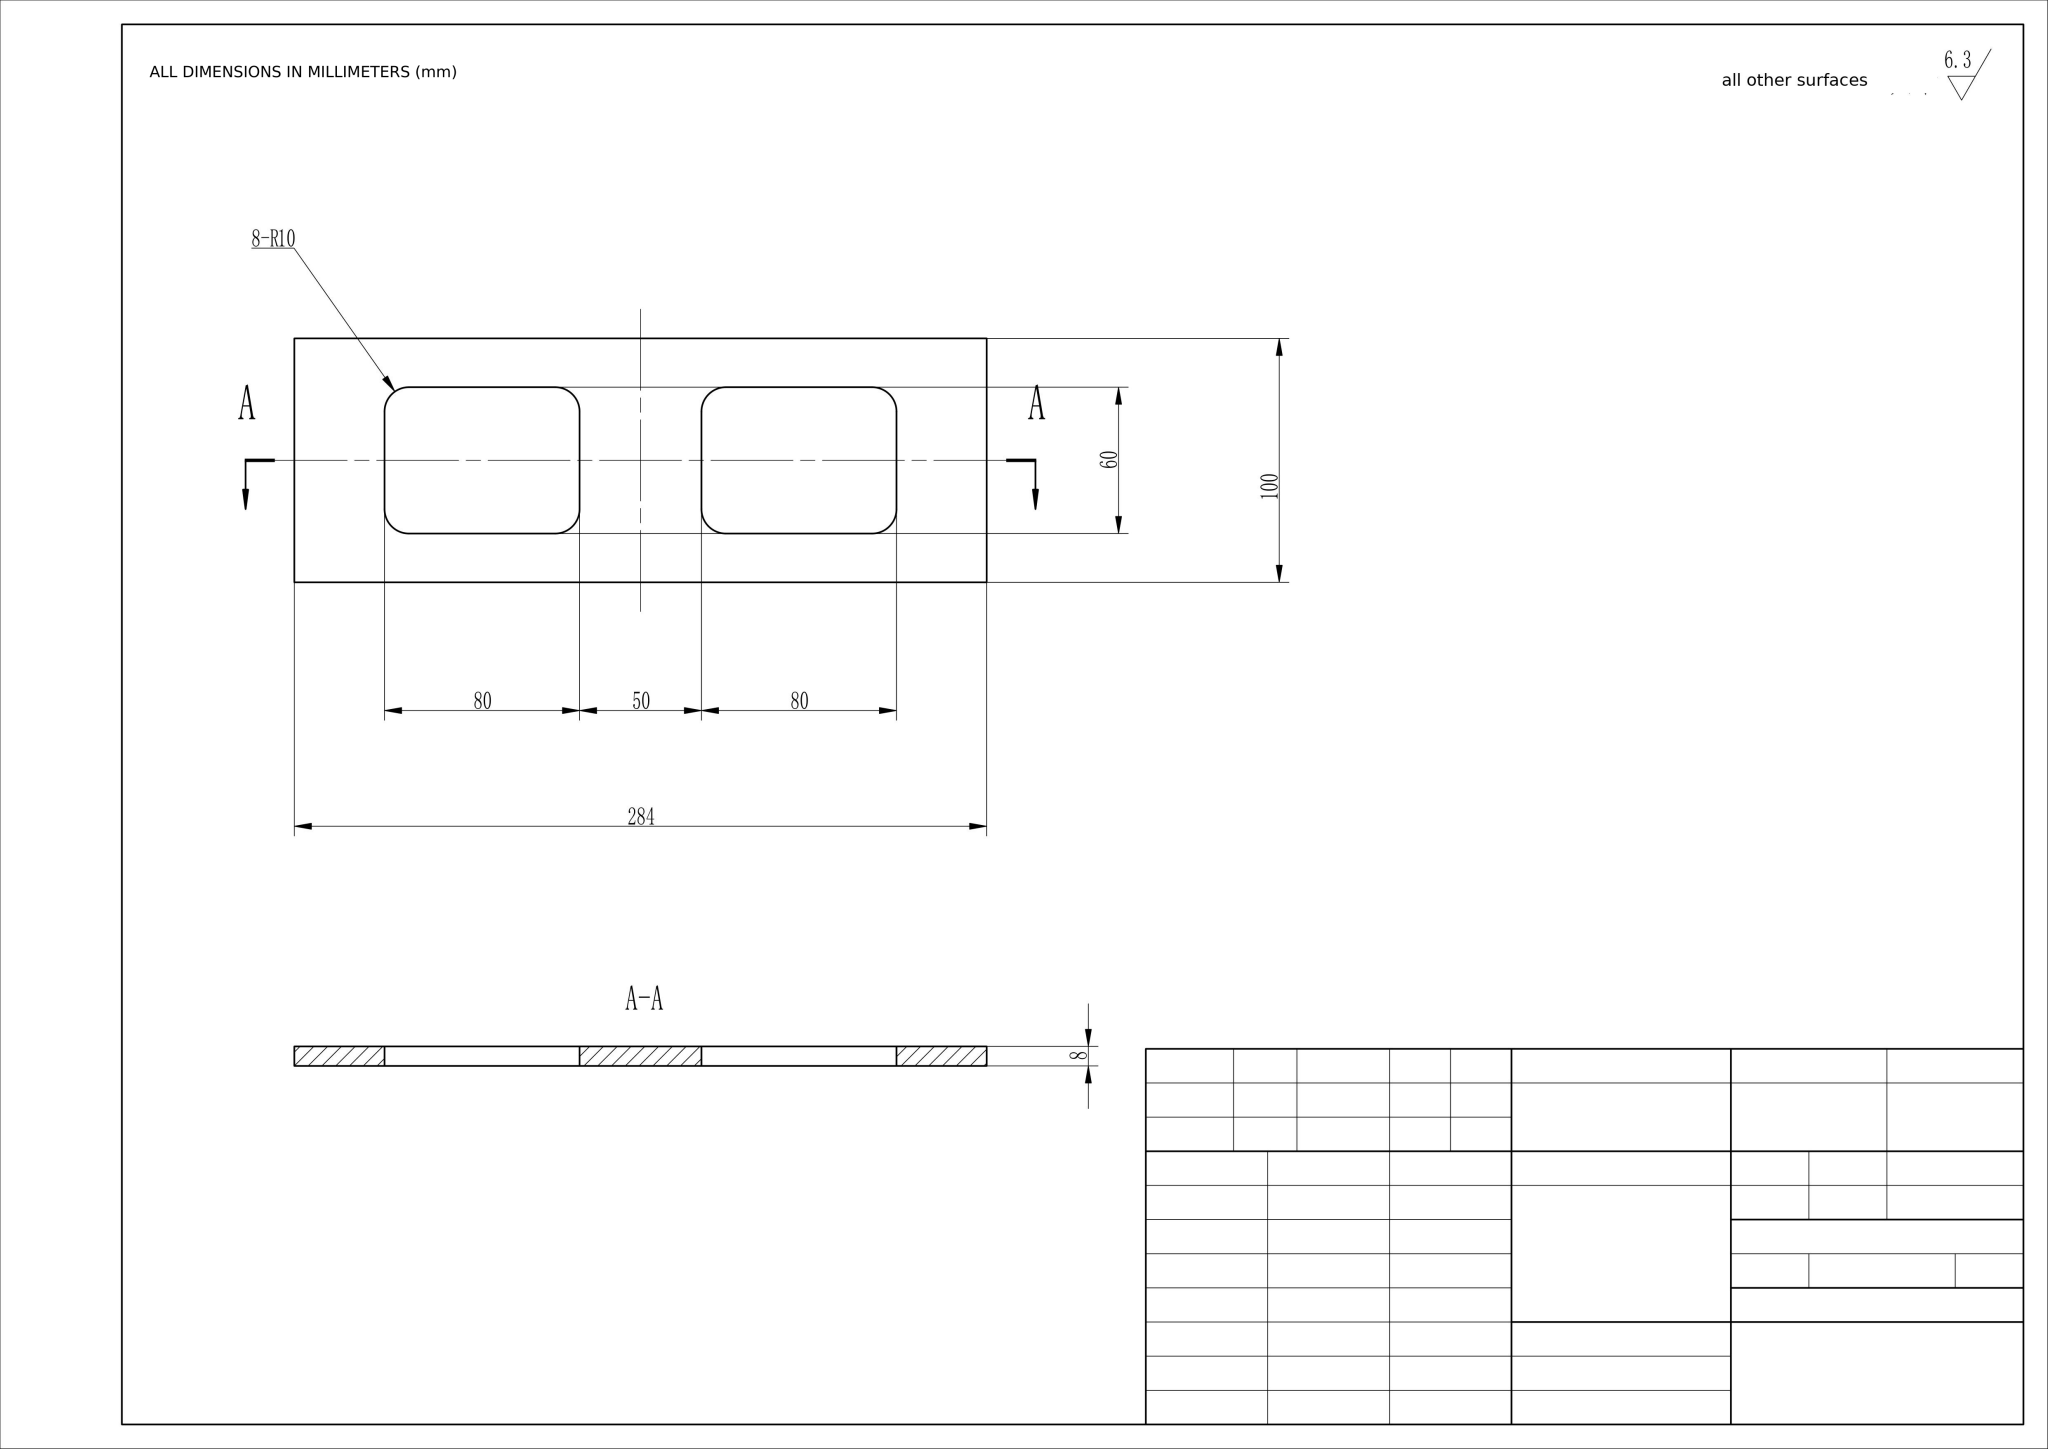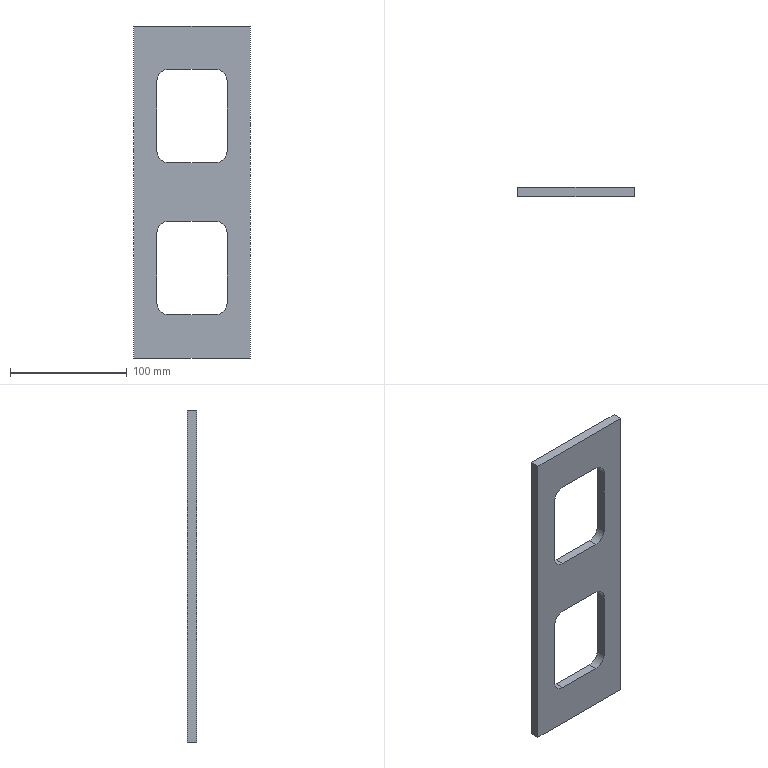Part | NX | mm | 1 solid | 22 faces | box 100 x 8 x 284 mm | volume 151773 mm3 | plane 14 | cylinder 8 | commonest cylinder face diameters 20 x8
STEP:
#1=CARTESIAN_POINT('',(0.,0.,0.));
#2=DIRECTION('',(0.,0.,1.));
#3=DIRECTION('',(1.,0.,0.));
#4=AXIS2_PLACEMENT_3D('',#1,#2,#3);
#5=(LENGTH_UNIT()NAMED_UNIT(*)SI_UNIT(.MILLI.,.METRE.));
#6=UNCERTAINTY_MEASURE_WITH_UNIT(LENGTH_MEASURE(0.00002),#5,'','');
#7=(NAMED_UNIT(*)PLANE_ANGLE_UNIT()SI_UNIT($,.RADIAN.));
#8=PLANE_ANGLE_MEASURE_WITH_UNIT(PLANE_ANGLE_MEASURE(0.01745),#7);
#9=DIMENSIONAL_EXPONENTS(0.,0.,0.,0.,0.,0.,0.);
#10=(CONVERSION_BASED_UNIT('',#8)NAMED_UNIT(#9)PLANE_ANGLE_UNIT());
#11=(NAMED_UNIT(*)SI_UNIT($,.STERADIAN.)SOLID_ANGLE_UNIT());
#12=(GEOMETRIC_REPRESENTATION_CONTEXT(3)GLOBAL_UNCERTAINTY_ASSIGNED_CONTEXT((#6))GLOBAL_UNIT_ASSIGNED_CONTEXT((#5,#10,#11))REPRESENTATION_CONTEXT('',''));
#13=SHAPE_REPRESENTATION('',(#4),#12);
#14=CARTESIAN_POINT('',(-0.,-8.,284.));
#15=VERTEX_POINT('',#14);
#16=CARTESIAN_POINT('',(0.,-8.,0.));
#17=VERTEX_POINT('',#16);
#18=CARTESIAN_POINT('',(-0.,-8.,284.));
#19=DIRECTION('',(0.,0.,-1.));
#20=VECTOR('',#19,1.);
#21=LINE('',#18,#20);
#22=EDGE_CURVE('',#15,#17,#21,.T.);
#23=ORIENTED_EDGE('',*,*,#22,.T.);
#24=CARTESIAN_POINT('',(100.,-8.,0.));
#25=VERTEX_POINT('',#24);
#26=CARTESIAN_POINT('',(0.,-8.,0.));
#27=DIRECTION('',(1.,0.,0.));
#28=VECTOR('',#27,1.);
#29=LINE('',#26,#28);
#30=EDGE_CURVE('',#17,#25,#29,.T.);
#31=ORIENTED_EDGE('',*,*,#30,.T.);
#32=CARTESIAN_POINT('',(100.,-8.,284.));
#33=VERTEX_POINT('',#32);
#34=CARTESIAN_POINT('',(100.,-8.,0.));
#35=DIRECTION('',(-0.,0.,1.));
#36=VECTOR('',#35,1.);
#37=LINE('',#34,#36);
#38=EDGE_CURVE('',#25,#33,#37,.T.);
#39=ORIENTED_EDGE('',*,*,#38,.T.);
#40=CARTESIAN_POINT('',(100.,-8.,284.));
#41=DIRECTION('',(-1.,0.,0.));
#42=VECTOR('',#41,1.);
#43=LINE('',#40,#42);
#44=EDGE_CURVE('',#33,#15,#43,.T.);
#45=ORIENTED_EDGE('',*,*,#44,.T.);
#46=EDGE_LOOP('',(#23,#31,#39,#45));
#47=FACE_BOUND('',#46,.T.);
#48=CARTESIAN_POINT('',(80.,-8.,237.));
#49=VERTEX_POINT('',#48);
#50=CARTESIAN_POINT('',(80.,-8.,177.));
#51=VERTEX_POINT('',#50);
#52=CARTESIAN_POINT('',(80.,-8.,247.));
#53=DIRECTION('',(0.,0.,-1.));
#54=VECTOR('',#53,1.);
#55=LINE('',#52,#54);
#56=EDGE_CURVE('',#49,#51,#55,.T.);
#57=ORIENTED_EDGE('',*,*,#56,.T.);
#58=CARTESIAN_POINT('',(70.,-8.,167.));
#59=VERTEX_POINT('',#58);
#60=CARTESIAN_POINT('',(70.,-8.,177.));
#61=DIRECTION('',(0.,1.,0.));
#62=DIRECTION('',(0.,0.,-1.));
#63=AXIS2_PLACEMENT_3D('',#60,#61,#62);
#64=CIRCLE('',#63,10.);
#65=EDGE_CURVE('',#51,#59,#64,.T.);
#66=ORIENTED_EDGE('',*,*,#65,.T.);
#67=CARTESIAN_POINT('',(30.,-8.,167.));
#68=VERTEX_POINT('',#67);
#69=CARTESIAN_POINT('',(80.,-8.,167.));
#70=DIRECTION('',(-1.,0.,0.));
#71=VECTOR('',#70,1.);
#72=LINE('',#69,#71);
#73=EDGE_CURVE('',#59,#68,#72,.T.);
#74=ORIENTED_EDGE('',*,*,#73,.T.);
#75=CARTESIAN_POINT('',(20.,-8.,177.));
#76=VERTEX_POINT('',#75);
#77=CARTESIAN_POINT('',(30.,-8.,177.));
#78=DIRECTION('',(0.,1.,0.));
#79=DIRECTION('',(0.,0.,-1.));
#80=AXIS2_PLACEMENT_3D('',#77,#78,#79);
#81=CIRCLE('',#80,10.);
#82=EDGE_CURVE('',#68,#76,#81,.T.);
#83=ORIENTED_EDGE('',*,*,#82,.T.);
#84=CARTESIAN_POINT('',(20.,-8.,237.));
#85=VERTEX_POINT('',#84);
#86=CARTESIAN_POINT('',(20.,-8.,167.));
#87=DIRECTION('',(0.,0.,1.));
#88=VECTOR('',#87,1.);
#89=LINE('',#86,#88);
#90=EDGE_CURVE('',#76,#85,#89,.T.);
#91=ORIENTED_EDGE('',*,*,#90,.T.);
#92=CARTESIAN_POINT('',(30.,-8.,247.));
#93=VERTEX_POINT('',#92);
#94=CARTESIAN_POINT('',(30.,-8.,237.));
#95=DIRECTION('',(0.,1.,0.));
#96=DIRECTION('',(0.,0.,-1.));
#97=AXIS2_PLACEMENT_3D('',#94,#95,#96);
#98=CIRCLE('',#97,10.);
#99=EDGE_CURVE('',#85,#93,#98,.T.);
#100=ORIENTED_EDGE('',*,*,#99,.T.);
#101=CARTESIAN_POINT('',(70.,-8.,247.));
#102=VERTEX_POINT('',#101);
#103=CARTESIAN_POINT('',(20.,-8.,247.));
#104=DIRECTION('',(1.,0.,0.));
#105=VECTOR('',#104,1.);
#106=LINE('',#103,#105);
#107=EDGE_CURVE('',#93,#102,#106,.T.);
#108=ORIENTED_EDGE('',*,*,#107,.T.);
#109=CARTESIAN_POINT('',(70.,-8.,237.));
#110=DIRECTION('',(0.,1.,0.));
#111=DIRECTION('',(0.,0.,-1.));
#112=AXIS2_PLACEMENT_3D('',#109,#110,#111);
#113=CIRCLE('',#112,10.);
#114=EDGE_CURVE('',#102,#49,#113,.T.);
#115=ORIENTED_EDGE('',*,*,#114,.T.);
#116=EDGE_LOOP('',(#57,#66,#74,#83,#91,#100,#108,#115));
#117=FACE_BOUND('',#116,.T.);
#118=CARTESIAN_POINT('',(80.,-8.,107.));
#119=VERTEX_POINT('',#118);
#120=CARTESIAN_POINT('',(80.,-8.,47.));
#121=VERTEX_POINT('',#120);
#122=CARTESIAN_POINT('',(80.,-8.,117.));
#123=DIRECTION('',(-0.,0.,-1.));
#124=VECTOR('',#123,1.);
#125=LINE('',#122,#124);
#126=EDGE_CURVE('',#119,#121,#125,.T.);
#127=ORIENTED_EDGE('',*,*,#126,.T.);
#128=CARTESIAN_POINT('',(70.,-8.,37.));
#129=VERTEX_POINT('',#128);
#130=CARTESIAN_POINT('',(70.,-8.,47.));
#131=DIRECTION('',(0.,1.,0.));
#132=DIRECTION('',(0.,0.,-1.));
#133=AXIS2_PLACEMENT_3D('',#130,#131,#132);
#134=CIRCLE('',#133,10.);
#135=EDGE_CURVE('',#121,#129,#134,.T.);
#136=ORIENTED_EDGE('',*,*,#135,.T.);
#137=CARTESIAN_POINT('',(30.,-8.,37.));
#138=VERTEX_POINT('',#137);
#139=CARTESIAN_POINT('',(80.,-8.,37.));
#140=DIRECTION('',(-1.,0.,0.));
#141=VECTOR('',#140,1.);
#142=LINE('',#139,#141);
#143=EDGE_CURVE('',#129,#138,#142,.T.);
#144=ORIENTED_EDGE('',*,*,#143,.T.);
#145=CARTESIAN_POINT('',(20.,-8.,47.));
#146=VERTEX_POINT('',#145);
#147=CARTESIAN_POINT('',(30.,-8.,47.));
#148=DIRECTION('',(0.,1.,0.));
#149=DIRECTION('',(0.,0.,-1.));
#150=AXIS2_PLACEMENT_3D('',#147,#148,#149);
#151=CIRCLE('',#150,10.);
#152=EDGE_CURVE('',#138,#146,#151,.T.);
#153=ORIENTED_EDGE('',*,*,#152,.T.);
#154=CARTESIAN_POINT('',(20.,-8.,107.));
#155=VERTEX_POINT('',#154);
#156=CARTESIAN_POINT('',(20.,-8.,37.));
#157=DIRECTION('',(-0.,0.,1.));
#158=VECTOR('',#157,1.);
#159=LINE('',#156,#158);
#160=EDGE_CURVE('',#146,#155,#159,.T.);
#161=ORIENTED_EDGE('',*,*,#160,.T.);
#162=CARTESIAN_POINT('',(30.,-8.,117.));
#163=VERTEX_POINT('',#162);
#164=CARTESIAN_POINT('',(30.,-8.,107.));
#165=DIRECTION('',(0.,1.,0.));
#166=DIRECTION('',(0.,0.,-1.));
#167=AXIS2_PLACEMENT_3D('',#164,#165,#166);
#168=CIRCLE('',#167,10.);
#169=EDGE_CURVE('',#155,#163,#168,.T.);
#170=ORIENTED_EDGE('',*,*,#169,.T.);
#171=CARTESIAN_POINT('',(70.,-8.,117.));
#172=VERTEX_POINT('',#171);
#173=CARTESIAN_POINT('',(20.,-8.,117.));
#174=DIRECTION('',(1.,0.,0.));
#175=VECTOR('',#174,1.);
#176=LINE('',#173,#175);
#177=EDGE_CURVE('',#163,#172,#176,.T.);
#178=ORIENTED_EDGE('',*,*,#177,.T.);
#179=CARTESIAN_POINT('',(70.,-8.,107.));
#180=DIRECTION('',(0.,1.,0.));
#181=DIRECTION('',(0.,0.,-1.));
#182=AXIS2_PLACEMENT_3D('',#179,#180,#181);
#183=CIRCLE('',#182,10.);
#184=EDGE_CURVE('',#172,#119,#183,.T.);
#185=ORIENTED_EDGE('',*,*,#184,.T.);
#186=EDGE_LOOP('',(#127,#136,#144,#153,#161,#170,#178,#185));
#187=FACE_BOUND('',#186,.T.);
#188=CARTESIAN_POINT('',(0.,-8.,0.));
#189=DIRECTION('',(0.,-1.,0.));
#190=DIRECTION('',(0.,0.,-1.));
#191=AXIS2_PLACEMENT_3D('',#188,#189,#190);
#192=PLANE('',#191);
#193=ADVANCED_FACE('',(#47,#117,#187),#192,.T.);
#194=CARTESIAN_POINT('',(20.,0.,177.));
#195=VERTEX_POINT('',#194);
#196=CARTESIAN_POINT('',(20.,0.,237.));
#197=VERTEX_POINT('',#196);
#198=CARTESIAN_POINT('',(20.,0.,167.));
#199=DIRECTION('',(0.,0.,1.));
#200=VECTOR('',#199,1.);
#201=LINE('',#198,#200);
#202=EDGE_CURVE('',#195,#197,#201,.T.);
#203=ORIENTED_EDGE('',*,*,#202,.F.);
#204=CARTESIAN_POINT('',(30.,0.,167.));
#205=VERTEX_POINT('',#204);
#206=CARTESIAN_POINT('',(30.,0.,177.));
#207=DIRECTION('',(0.,-1.,0.));
#208=DIRECTION('',(0.,0.,-1.));
#209=AXIS2_PLACEMENT_3D('',#206,#207,#208);
#210=CIRCLE('',#209,10.);
#211=EDGE_CURVE('',#195,#205,#210,.T.);
#212=ORIENTED_EDGE('',*,*,#211,.T.);
#213=CARTESIAN_POINT('',(70.,0.,167.));
#214=VERTEX_POINT('',#213);
#215=CARTESIAN_POINT('',(80.,0.,167.));
#216=DIRECTION('',(-1.,0.,0.));
#217=VECTOR('',#216,1.);
#218=LINE('',#215,#217);
#219=EDGE_CURVE('',#214,#205,#218,.T.);
#220=ORIENTED_EDGE('',*,*,#219,.F.);
#221=CARTESIAN_POINT('',(80.,0.,177.));
#222=VERTEX_POINT('',#221);
#223=CARTESIAN_POINT('',(70.,0.,177.));
#224=DIRECTION('',(0.,-1.,0.));
#225=DIRECTION('',(0.,0.,-1.));
#226=AXIS2_PLACEMENT_3D('',#223,#224,#225);
#227=CIRCLE('',#226,10.);
#228=EDGE_CURVE('',#214,#222,#227,.T.);
#229=ORIENTED_EDGE('',*,*,#228,.T.);
#230=CARTESIAN_POINT('',(80.,0.,237.));
#231=VERTEX_POINT('',#230);
#232=CARTESIAN_POINT('',(80.,0.,247.));
#233=DIRECTION('',(0.,0.,-1.));
#234=VECTOR('',#233,1.);
#235=LINE('',#232,#234);
#236=EDGE_CURVE('',#231,#222,#235,.T.);
#237=ORIENTED_EDGE('',*,*,#236,.F.);
#238=CARTESIAN_POINT('',(70.,0.,247.));
#239=VERTEX_POINT('',#238);
#240=CARTESIAN_POINT('',(70.,0.,237.));
#241=DIRECTION('',(0.,-1.,0.));
#242=DIRECTION('',(0.,0.,-1.));
#243=AXIS2_PLACEMENT_3D('',#240,#241,#242);
#244=CIRCLE('',#243,10.);
#245=EDGE_CURVE('',#231,#239,#244,.T.);
#246=ORIENTED_EDGE('',*,*,#245,.T.);
#247=CARTESIAN_POINT('',(30.,0.,247.));
#248=VERTEX_POINT('',#247);
#249=CARTESIAN_POINT('',(20.,0.,247.));
#250=DIRECTION('',(1.,0.,0.));
#251=VECTOR('',#250,1.);
#252=LINE('',#249,#251);
#253=EDGE_CURVE('',#248,#239,#252,.T.);
#254=ORIENTED_EDGE('',*,*,#253,.F.);
#255=CARTESIAN_POINT('',(30.,0.,237.));
#256=DIRECTION('',(0.,-1.,0.));
#257=DIRECTION('',(0.,0.,-1.));
#258=AXIS2_PLACEMENT_3D('',#255,#256,#257);
#259=CIRCLE('',#258,10.);
#260=EDGE_CURVE('',#248,#197,#259,.T.);
#261=ORIENTED_EDGE('',*,*,#260,.T.);
#262=EDGE_LOOP('',(#203,#212,#220,#229,#237,#246,#254,#261));
#263=FACE_BOUND('',#262,.T.);
#264=CARTESIAN_POINT('',(-0.,0.,284.));
#265=VERTEX_POINT('',#264);
#266=CARTESIAN_POINT('',(0.,0.,0.));
#267=VERTEX_POINT('',#266);
#268=CARTESIAN_POINT('',(-0.,0.,284.));
#269=DIRECTION('',(0.,0.,-1.));
#270=VECTOR('',#269,1.);
#271=LINE('',#268,#270);
#272=EDGE_CURVE('',#265,#267,#271,.T.);
#273=ORIENTED_EDGE('',*,*,#272,.F.);
#274=CARTESIAN_POINT('',(100.,0.,284.));
#275=VERTEX_POINT('',#274);
#276=CARTESIAN_POINT('',(100.,0.,284.));
#277=DIRECTION('',(-1.,0.,0.));
#278=VECTOR('',#277,1.);
#279=LINE('',#276,#278);
#280=EDGE_CURVE('',#275,#265,#279,.T.);
#281=ORIENTED_EDGE('',*,*,#280,.F.);
#282=CARTESIAN_POINT('',(100.,0.,0.));
#283=VERTEX_POINT('',#282);
#284=CARTESIAN_POINT('',(100.,0.,0.));
#285=DIRECTION('',(-0.,0.,1.));
#286=VECTOR('',#285,1.);
#287=LINE('',#284,#286);
#288=EDGE_CURVE('',#283,#275,#287,.T.);
#289=ORIENTED_EDGE('',*,*,#288,.F.);
#290=CARTESIAN_POINT('',(0.,0.,0.));
#291=DIRECTION('',(1.,0.,0.));
#292=VECTOR('',#291,1.);
#293=LINE('',#290,#292);
#294=EDGE_CURVE('',#267,#283,#293,.T.);
#295=ORIENTED_EDGE('',*,*,#294,.F.);
#296=EDGE_LOOP('',(#273,#281,#289,#295));
#297=FACE_BOUND('',#296,.T.);
#298=CARTESIAN_POINT('',(20.,0.,47.));
#299=VERTEX_POINT('',#298);
#300=CARTESIAN_POINT('',(20.,0.,107.));
#301=VERTEX_POINT('',#300);
#302=CARTESIAN_POINT('',(20.,0.,37.));
#303=DIRECTION('',(-0.,0.,1.));
#304=VECTOR('',#303,1.);
#305=LINE('',#302,#304);
#306=EDGE_CURVE('',#299,#301,#305,.T.);
#307=ORIENTED_EDGE('',*,*,#306,.F.);
#308=CARTESIAN_POINT('',(30.,0.,37.));
#309=VERTEX_POINT('',#308);
#310=CARTESIAN_POINT('',(30.,0.,47.));
#311=DIRECTION('',(0.,-1.,0.));
#312=DIRECTION('',(0.,0.,-1.));
#313=AXIS2_PLACEMENT_3D('',#310,#311,#312);
#314=CIRCLE('',#313,10.);
#315=EDGE_CURVE('',#299,#309,#314,.T.);
#316=ORIENTED_EDGE('',*,*,#315,.T.);
#317=CARTESIAN_POINT('',(70.,0.,37.));
#318=VERTEX_POINT('',#317);
#319=CARTESIAN_POINT('',(80.,0.,37.));
#320=DIRECTION('',(-1.,0.,0.));
#321=VECTOR('',#320,1.);
#322=LINE('',#319,#321);
#323=EDGE_CURVE('',#318,#309,#322,.T.);
#324=ORIENTED_EDGE('',*,*,#323,.F.);
#325=CARTESIAN_POINT('',(80.,0.,47.));
#326=VERTEX_POINT('',#325);
#327=CARTESIAN_POINT('',(70.,0.,47.));
#328=DIRECTION('',(0.,-1.,0.));
#329=DIRECTION('',(0.,0.,-1.));
#330=AXIS2_PLACEMENT_3D('',#327,#328,#329);
#331=CIRCLE('',#330,10.);
#332=EDGE_CURVE('',#318,#326,#331,.T.);
#333=ORIENTED_EDGE('',*,*,#332,.T.);
#334=CARTESIAN_POINT('',(80.,0.,107.));
#335=VERTEX_POINT('',#334);
#336=CARTESIAN_POINT('',(80.,0.,117.));
#337=DIRECTION('',(-0.,0.,-1.));
#338=VECTOR('',#337,1.);
#339=LINE('',#336,#338);
#340=EDGE_CURVE('',#335,#326,#339,.T.);
#341=ORIENTED_EDGE('',*,*,#340,.F.);
#342=CARTESIAN_POINT('',(70.,0.,117.));
#343=VERTEX_POINT('',#342);
#344=CARTESIAN_POINT('',(70.,0.,107.));
#345=DIRECTION('',(0.,-1.,0.));
#346=DIRECTION('',(0.,0.,-1.));
#347=AXIS2_PLACEMENT_3D('',#344,#345,#346);
#348=CIRCLE('',#347,10.);
#349=EDGE_CURVE('',#335,#343,#348,.T.);
#350=ORIENTED_EDGE('',*,*,#349,.T.);
#351=CARTESIAN_POINT('',(30.,0.,117.));
#352=VERTEX_POINT('',#351);
#353=CARTESIAN_POINT('',(20.,0.,117.));
#354=DIRECTION('',(1.,0.,0.));
#355=VECTOR('',#354,1.);
#356=LINE('',#353,#355);
#357=EDGE_CURVE('',#352,#343,#356,.T.);
#358=ORIENTED_EDGE('',*,*,#357,.F.);
#359=CARTESIAN_POINT('',(30.,0.,107.));
#360=DIRECTION('',(0.,-1.,0.));
#361=DIRECTION('',(0.,0.,-1.));
#362=AXIS2_PLACEMENT_3D('',#359,#360,#361);
#363=CIRCLE('',#362,10.);
#364=EDGE_CURVE('',#352,#301,#363,.T.);
#365=ORIENTED_EDGE('',*,*,#364,.T.);
#366=EDGE_LOOP('',(#307,#316,#324,#333,#341,#350,#358,#365));
#367=FACE_BOUND('',#366,.T.);
#368=CARTESIAN_POINT('',(0.,0.,0.));
#369=DIRECTION('',(0.,-1.,0.));
#370=DIRECTION('',(0.,0.,-1.));
#371=AXIS2_PLACEMENT_3D('',#368,#369,#370);
#372=PLANE('',#371);
#373=ADVANCED_FACE('',(#263,#297,#367),#372,.F.);
#374=ORIENTED_EDGE('',*,*,#272,.T.);
#375=CARTESIAN_POINT('',(0.,-8.,0.));
#376=DIRECTION('',(0.,1.,0.));
#377=VECTOR('',#376,1.);
#378=LINE('',#375,#377);
#379=EDGE_CURVE('',#17,#267,#378,.T.);
#380=ORIENTED_EDGE('',*,*,#379,.F.);
#381=ORIENTED_EDGE('',*,*,#22,.F.);
#382=CARTESIAN_POINT('',(-0.,-8.,284.));
#383=DIRECTION('',(0.,1.,0.));
#384=VECTOR('',#383,1.);
#385=LINE('',#382,#384);
#386=EDGE_CURVE('',#15,#265,#385,.T.);
#387=ORIENTED_EDGE('',*,*,#386,.T.);
#388=EDGE_LOOP('',(#374,#380,#381,#387));
#389=FACE_OUTER_BOUND('',#388,.T.);
#390=CARTESIAN_POINT('',(-0.,-8.,284.));
#391=DIRECTION('',(1.,0.,0.));
#392=DIRECTION('',(0.,0.,-1.));
#393=AXIS2_PLACEMENT_3D('',#390,#391,#392);
#394=PLANE('',#393);
#395=ADVANCED_FACE('',(#389),#394,.F.);
#396=ORIENTED_EDGE('',*,*,#294,.T.);
#397=CARTESIAN_POINT('',(100.,-8.,0.));
#398=DIRECTION('',(0.,1.,0.));
#399=VECTOR('',#398,1.);
#400=LINE('',#397,#399);
#401=EDGE_CURVE('',#25,#283,#400,.T.);
#402=ORIENTED_EDGE('',*,*,#401,.F.);
#403=ORIENTED_EDGE('',*,*,#30,.F.);
#404=ORIENTED_EDGE('',*,*,#379,.T.);
#405=EDGE_LOOP('',(#396,#402,#403,#404));
#406=FACE_OUTER_BOUND('',#405,.T.);
#407=CARTESIAN_POINT('',(0.,-8.,0.));
#408=DIRECTION('',(0.,0.,1.));
#409=DIRECTION('',(1.,0.,0.));
#410=AXIS2_PLACEMENT_3D('',#407,#408,#409);
#411=PLANE('',#410);
#412=ADVANCED_FACE('',(#406),#411,.F.);
#413=ORIENTED_EDGE('',*,*,#288,.T.);
#414=CARTESIAN_POINT('',(100.,-8.,284.));
#415=DIRECTION('',(0.,1.,0.));
#416=VECTOR('',#415,1.);
#417=LINE('',#414,#416);
#418=EDGE_CURVE('',#33,#275,#417,.T.);
#419=ORIENTED_EDGE('',*,*,#418,.F.);
#420=ORIENTED_EDGE('',*,*,#38,.F.);
#421=ORIENTED_EDGE('',*,*,#401,.T.);
#422=EDGE_LOOP('',(#413,#419,#420,#421));
#423=FACE_OUTER_BOUND('',#422,.T.);
#424=CARTESIAN_POINT('',(100.,-8.,0.));
#425=DIRECTION('',(-1.,0.,-0.));
#426=DIRECTION('',(-0.,0.,1.));
#427=AXIS2_PLACEMENT_3D('',#424,#425,#426);
#428=PLANE('',#427);
#429=ADVANCED_FACE('',(#423),#428,.F.);
#430=ORIENTED_EDGE('',*,*,#280,.T.);
#431=ORIENTED_EDGE('',*,*,#386,.F.);
#432=ORIENTED_EDGE('',*,*,#44,.F.);
#433=ORIENTED_EDGE('',*,*,#418,.T.);
#434=EDGE_LOOP('',(#430,#431,#432,#433));
#435=FACE_OUTER_BOUND('',#434,.T.);
#436=CARTESIAN_POINT('',(100.,-8.,284.));
#437=DIRECTION('',(0.,0.,-1.));
#438=DIRECTION('',(-1.,0.,0.));
#439=AXIS2_PLACEMENT_3D('',#436,#437,#438);
#440=PLANE('',#439);
#441=ADVANCED_FACE('',(#435),#440,.F.);
#442=ORIENTED_EDGE('',*,*,#90,.F.);
#443=CARTESIAN_POINT('',(20.,0.,177.));
#444=DIRECTION('',(0.,1.,0.));
#445=VECTOR('',#444,1.);
#446=LINE('',#443,#445);
#447=EDGE_CURVE('',#76,#195,#446,.T.);
#448=ORIENTED_EDGE('',*,*,#447,.T.);
#449=ORIENTED_EDGE('',*,*,#202,.T.);
#450=CARTESIAN_POINT('',(20.,-8.,237.));
#451=DIRECTION('',(0.,-1.,0.));
#452=VECTOR('',#451,1.);
#453=LINE('',#450,#452);
#454=EDGE_CURVE('',#197,#85,#453,.T.);
#455=ORIENTED_EDGE('',*,*,#454,.T.);
#456=EDGE_LOOP('',(#442,#448,#449,#455));
#457=FACE_OUTER_BOUND('',#456,.T.);
#458=CARTESIAN_POINT('',(20.,-8.,167.));
#459=DIRECTION('',(-1.,0.,0.));
#460=DIRECTION('',(0.,0.,1.));
#461=AXIS2_PLACEMENT_3D('',#458,#459,#460);
#462=PLANE('',#461);
#463=ADVANCED_FACE('',(#457),#462,.F.);
#464=ORIENTED_EDGE('',*,*,#253,.T.);
#465=CARTESIAN_POINT('',(70.,-8.,247.));
#466=DIRECTION('',(0.,-1.,0.));
#467=VECTOR('',#466,1.);
#468=LINE('',#465,#467);
#469=EDGE_CURVE('',#239,#102,#468,.T.);
#470=ORIENTED_EDGE('',*,*,#469,.T.);
#471=ORIENTED_EDGE('',*,*,#107,.F.);
#472=CARTESIAN_POINT('',(30.,0.,247.));
#473=DIRECTION('',(0.,1.,0.));
#474=VECTOR('',#473,1.);
#475=LINE('',#472,#474);
#476=EDGE_CURVE('',#93,#248,#475,.T.);
#477=ORIENTED_EDGE('',*,*,#476,.T.);
#478=EDGE_LOOP('',(#464,#470,#471,#477));
#479=FACE_OUTER_BOUND('',#478,.T.);
#480=CARTESIAN_POINT('',(20.,-8.,247.));
#481=DIRECTION('',(0.,0.,1.));
#482=DIRECTION('',(1.,0.,0.));
#483=AXIS2_PLACEMENT_3D('',#480,#481,#482);
#484=PLANE('',#483);
#485=ADVANCED_FACE('',(#479),#484,.F.);
#486=ORIENTED_EDGE('',*,*,#236,.T.);
#487=CARTESIAN_POINT('',(80.,-8.,177.));
#488=DIRECTION('',(0.,-1.,0.));
#489=VECTOR('',#488,1.);
#490=LINE('',#487,#489);
#491=EDGE_CURVE('',#222,#51,#490,.T.);
#492=ORIENTED_EDGE('',*,*,#491,.T.);
#493=ORIENTED_EDGE('',*,*,#56,.F.);
#494=CARTESIAN_POINT('',(80.,0.,237.));
#495=DIRECTION('',(0.,1.,0.));
#496=VECTOR('',#495,1.);
#497=LINE('',#494,#496);
#498=EDGE_CURVE('',#49,#231,#497,.T.);
#499=ORIENTED_EDGE('',*,*,#498,.T.);
#500=EDGE_LOOP('',(#486,#492,#493,#499));
#501=FACE_OUTER_BOUND('',#500,.T.);
#502=CARTESIAN_POINT('',(80.,-8.,247.));
#503=DIRECTION('',(1.,0.,0.));
#504=DIRECTION('',(0.,0.,-1.));
#505=AXIS2_PLACEMENT_3D('',#502,#503,#504);
#506=PLANE('',#505);
#507=ADVANCED_FACE('',(#501),#506,.F.);
#508=ORIENTED_EDGE('',*,*,#73,.F.);
#509=CARTESIAN_POINT('',(70.,0.,167.));
#510=DIRECTION('',(0.,1.,0.));
#511=VECTOR('',#510,1.);
#512=LINE('',#509,#511);
#513=EDGE_CURVE('',#59,#214,#512,.T.);
#514=ORIENTED_EDGE('',*,*,#513,.T.);
#515=ORIENTED_EDGE('',*,*,#219,.T.);
#516=CARTESIAN_POINT('',(30.,-8.,167.));
#517=DIRECTION('',(0.,-1.,0.));
#518=VECTOR('',#517,1.);
#519=LINE('',#516,#518);
#520=EDGE_CURVE('',#205,#68,#519,.T.);
#521=ORIENTED_EDGE('',*,*,#520,.T.);
#522=EDGE_LOOP('',(#508,#514,#515,#521));
#523=FACE_OUTER_BOUND('',#522,.T.);
#524=CARTESIAN_POINT('',(80.,-8.,167.));
#525=DIRECTION('',(-0.,0.,-1.));
#526=DIRECTION('',(-1.,0.,0.));
#527=AXIS2_PLACEMENT_3D('',#524,#525,#526);
#528=PLANE('',#527);
#529=ADVANCED_FACE('',(#523),#528,.F.);
#530=ORIENTED_EDGE('',*,*,#160,.F.);
#531=CARTESIAN_POINT('',(20.,0.,47.));
#532=DIRECTION('',(0.,1.,0.));
#533=VECTOR('',#532,1.);
#534=LINE('',#531,#533);
#535=EDGE_CURVE('',#146,#299,#534,.T.);
#536=ORIENTED_EDGE('',*,*,#535,.T.);
#537=ORIENTED_EDGE('',*,*,#306,.T.);
#538=CARTESIAN_POINT('',(20.,-8.,107.));
#539=DIRECTION('',(0.,-1.,0.));
#540=VECTOR('',#539,1.);
#541=LINE('',#538,#540);
#542=EDGE_CURVE('',#301,#155,#541,.T.);
#543=ORIENTED_EDGE('',*,*,#542,.T.);
#544=EDGE_LOOP('',(#530,#536,#537,#543));
#545=FACE_OUTER_BOUND('',#544,.T.);
#546=CARTESIAN_POINT('',(20.,-8.,37.));
#547=DIRECTION('',(-1.,0.,-0.));
#548=DIRECTION('',(-0.,0.,1.));
#549=AXIS2_PLACEMENT_3D('',#546,#547,#548);
#550=PLANE('',#549);
#551=ADVANCED_FACE('',(#545),#550,.F.);
#552=ORIENTED_EDGE('',*,*,#357,.T.);
#553=CARTESIAN_POINT('',(70.,-8.,117.));
#554=DIRECTION('',(0.,-1.,0.));
#555=VECTOR('',#554,1.);
#556=LINE('',#553,#555);
#557=EDGE_CURVE('',#343,#172,#556,.T.);
#558=ORIENTED_EDGE('',*,*,#557,.T.);
#559=ORIENTED_EDGE('',*,*,#177,.F.);
#560=CARTESIAN_POINT('',(30.,0.,117.));
#561=DIRECTION('',(0.,1.,0.));
#562=VECTOR('',#561,1.);
#563=LINE('',#560,#562);
#564=EDGE_CURVE('',#163,#352,#563,.T.);
#565=ORIENTED_EDGE('',*,*,#564,.T.);
#566=EDGE_LOOP('',(#552,#558,#559,#565));
#567=FACE_OUTER_BOUND('',#566,.T.);
#568=CARTESIAN_POINT('',(20.,-8.,117.));
#569=DIRECTION('',(0.,0.,1.));
#570=DIRECTION('',(1.,0.,0.));
#571=AXIS2_PLACEMENT_3D('',#568,#569,#570);
#572=PLANE('',#571);
#573=ADVANCED_FACE('',(#567),#572,.F.);
#574=ORIENTED_EDGE('',*,*,#126,.F.);
#575=CARTESIAN_POINT('',(80.,0.,107.));
#576=DIRECTION('',(0.,1.,0.));
#577=VECTOR('',#576,1.);
#578=LINE('',#575,#577);
#579=EDGE_CURVE('',#119,#335,#578,.T.);
#580=ORIENTED_EDGE('',*,*,#579,.T.);
#581=ORIENTED_EDGE('',*,*,#340,.T.);
#582=CARTESIAN_POINT('',(80.,-8.,47.));
#583=DIRECTION('',(0.,-1.,0.));
#584=VECTOR('',#583,1.);
#585=LINE('',#582,#584);
#586=EDGE_CURVE('',#326,#121,#585,.T.);
#587=ORIENTED_EDGE('',*,*,#586,.T.);
#588=EDGE_LOOP('',(#574,#580,#581,#587));
#589=FACE_OUTER_BOUND('',#588,.T.);
#590=CARTESIAN_POINT('',(80.,-8.,117.));
#591=DIRECTION('',(1.,0.,-0.));
#592=DIRECTION('',(-0.,0.,-1.));
#593=AXIS2_PLACEMENT_3D('',#590,#591,#592);
#594=PLANE('',#593);
#595=ADVANCED_FACE('',(#589),#594,.F.);
#596=ORIENTED_EDGE('',*,*,#143,.F.);
#597=CARTESIAN_POINT('',(70.,0.,37.));
#598=DIRECTION('',(0.,1.,0.));
#599=VECTOR('',#598,1.);
#600=LINE('',#597,#599);
#601=EDGE_CURVE('',#129,#318,#600,.T.);
#602=ORIENTED_EDGE('',*,*,#601,.T.);
#603=ORIENTED_EDGE('',*,*,#323,.T.);
#604=CARTESIAN_POINT('',(30.,-8.,37.));
#605=DIRECTION('',(0.,-1.,0.));
#606=VECTOR('',#605,1.);
#607=LINE('',#604,#606);
#608=EDGE_CURVE('',#309,#138,#607,.T.);
#609=ORIENTED_EDGE('',*,*,#608,.T.);
#610=EDGE_LOOP('',(#596,#602,#603,#609));
#611=FACE_OUTER_BOUND('',#610,.T.);
#612=CARTESIAN_POINT('',(80.,-8.,37.));
#613=DIRECTION('',(0.,0.,-1.));
#614=DIRECTION('',(-1.,0.,0.));
#615=AXIS2_PLACEMENT_3D('',#612,#613,#614);
#616=PLANE('',#615);
#617=ADVANCED_FACE('',(#611),#616,.F.);
#618=ORIENTED_EDGE('',*,*,#228,.F.);
#619=ORIENTED_EDGE('',*,*,#513,.F.);
#620=ORIENTED_EDGE('',*,*,#65,.F.);
#621=ORIENTED_EDGE('',*,*,#491,.F.);
#622=EDGE_LOOP('',(#618,#619,#620,#621));
#623=FACE_OUTER_BOUND('',#622,.T.);
#624=CARTESIAN_POINT('',(70.,-8.,177.));
#625=DIRECTION('',(0.,1.,0.));
#626=DIRECTION('',(0.,0.,1.));
#627=AXIS2_PLACEMENT_3D('',#624,#625,#626);
#628=CYLINDRICAL_SURFACE('',#627,10.);
#629=ADVANCED_FACE('',(#623),#628,.F.);
#630=ORIENTED_EDGE('',*,*,#245,.F.);
#631=ORIENTED_EDGE('',*,*,#498,.F.);
#632=ORIENTED_EDGE('',*,*,#114,.F.);
#633=ORIENTED_EDGE('',*,*,#469,.F.);
#634=EDGE_LOOP('',(#630,#631,#632,#633));
#635=FACE_OUTER_BOUND('',#634,.T.);
#636=CARTESIAN_POINT('',(70.,-8.,237.));
#637=DIRECTION('',(0.,1.,0.));
#638=DIRECTION('',(0.,0.,1.));
#639=AXIS2_PLACEMENT_3D('',#636,#637,#638);
#640=CYLINDRICAL_SURFACE('',#639,10.);
#641=ADVANCED_FACE('',(#635),#640,.F.);
#642=ORIENTED_EDGE('',*,*,#349,.F.);
#643=ORIENTED_EDGE('',*,*,#579,.F.);
#644=ORIENTED_EDGE('',*,*,#184,.F.);
#645=ORIENTED_EDGE('',*,*,#557,.F.);
#646=EDGE_LOOP('',(#642,#643,#644,#645));
#647=FACE_OUTER_BOUND('',#646,.T.);
#648=CARTESIAN_POINT('',(70.,-8.,107.));
#649=DIRECTION('',(0.,1.,0.));
#650=DIRECTION('',(0.,0.,1.));
#651=AXIS2_PLACEMENT_3D('',#648,#649,#650);
#652=CYLINDRICAL_SURFACE('',#651,10.);
#653=ADVANCED_FACE('',(#647),#652,.F.);
#654=ORIENTED_EDGE('',*,*,#332,.F.);
#655=ORIENTED_EDGE('',*,*,#601,.F.);
#656=ORIENTED_EDGE('',*,*,#135,.F.);
#657=ORIENTED_EDGE('',*,*,#586,.F.);
#658=EDGE_LOOP('',(#654,#655,#656,#657));
#659=FACE_OUTER_BOUND('',#658,.T.);
#660=CARTESIAN_POINT('',(70.,-8.,47.));
#661=DIRECTION('',(0.,1.,0.));
#662=DIRECTION('',(0.,0.,1.));
#663=AXIS2_PLACEMENT_3D('',#660,#661,#662);
#664=CYLINDRICAL_SURFACE('',#663,10.);
#665=ADVANCED_FACE('',(#659),#664,.F.);
#666=ORIENTED_EDGE('',*,*,#315,.F.);
#667=ORIENTED_EDGE('',*,*,#535,.F.);
#668=ORIENTED_EDGE('',*,*,#152,.F.);
#669=ORIENTED_EDGE('',*,*,#608,.F.);
#670=EDGE_LOOP('',(#666,#667,#668,#669));
#671=FACE_OUTER_BOUND('',#670,.T.);
#672=CARTESIAN_POINT('',(30.,-8.,47.));
#673=DIRECTION('',(0.,1.,0.));
#674=DIRECTION('',(0.,0.,1.));
#675=AXIS2_PLACEMENT_3D('',#672,#673,#674);
#676=CYLINDRICAL_SURFACE('',#675,10.);
#677=ADVANCED_FACE('',(#671),#676,.F.);
#678=ORIENTED_EDGE('',*,*,#211,.F.);
#679=ORIENTED_EDGE('',*,*,#447,.F.);
#680=ORIENTED_EDGE('',*,*,#82,.F.);
#681=ORIENTED_EDGE('',*,*,#520,.F.);
#682=EDGE_LOOP('',(#678,#679,#680,#681));
#683=FACE_OUTER_BOUND('',#682,.T.);
#684=CARTESIAN_POINT('',(30.,-8.,177.));
#685=DIRECTION('',(0.,1.,0.));
#686=DIRECTION('',(0.,0.,1.));
#687=AXIS2_PLACEMENT_3D('',#684,#685,#686);
#688=CYLINDRICAL_SURFACE('',#687,10.);
#689=ADVANCED_FACE('',(#683),#688,.F.);
#690=ORIENTED_EDGE('',*,*,#364,.F.);
#691=ORIENTED_EDGE('',*,*,#564,.F.);
#692=ORIENTED_EDGE('',*,*,#169,.F.);
#693=ORIENTED_EDGE('',*,*,#542,.F.);
#694=EDGE_LOOP('',(#690,#691,#692,#693));
#695=FACE_OUTER_BOUND('',#694,.T.);
#696=CARTESIAN_POINT('',(30.,-8.,107.));
#697=DIRECTION('',(0.,1.,0.));
#698=DIRECTION('',(0.,0.,1.));
#699=AXIS2_PLACEMENT_3D('',#696,#697,#698);
#700=CYLINDRICAL_SURFACE('',#699,10.);
#701=ADVANCED_FACE('',(#695),#700,.F.);
#702=ORIENTED_EDGE('',*,*,#260,.F.);
#703=ORIENTED_EDGE('',*,*,#476,.F.);
#704=ORIENTED_EDGE('',*,*,#99,.F.);
#705=ORIENTED_EDGE('',*,*,#454,.F.);
#706=EDGE_LOOP('',(#702,#703,#704,#705));
#707=FACE_OUTER_BOUND('',#706,.T.);
#708=CARTESIAN_POINT('',(30.,-8.,237.));
#709=DIRECTION('',(0.,1.,0.));
#710=DIRECTION('',(0.,0.,1.));
#711=AXIS2_PLACEMENT_3D('',#708,#709,#710);
#712=CYLINDRICAL_SURFACE('',#711,10.);
#713=ADVANCED_FACE('',(#707),#712,.F.);
#714=CLOSED_SHELL('',(#193,#373,#395,#412,#429,#441,#463,#485,#507,#529,#551,#573,#595,#617,#629,#641,#653,#665,#677,#689,#701,#713));
#715=MANIFOLD_SOLID_BREP('',#714);
#716=ADVANCED_BREP_SHAPE_REPRESENTATION('',(#715),#12);
#717=SHAPE_REPRESENTATION_RELATIONSHIP('','',#13,#716);
#718=PRESENTATION_LAYER_ASSIGNMENT('','',(#715));
#719=COLOUR_RGB('',1.,0.6,0.);
#720=FILL_AREA_STYLE_COLOUR('',#719);
#721=FILL_AREA_STYLE('',(#720));
#722=SURFACE_STYLE_FILL_AREA(#721);
#723=SURFACE_SIDE_STYLE('',(#722));
#724=SURFACE_STYLE_USAGE(.BOTH.,#723);
#725=PRESENTATION_STYLE_ASSIGNMENT((#724));
#726=STYLED_ITEM('',(#725),#715);
#727=MECHANICAL_DESIGN_GEOMETRIC_PRESENTATION_REPRESENTATION('',(#726),#12);